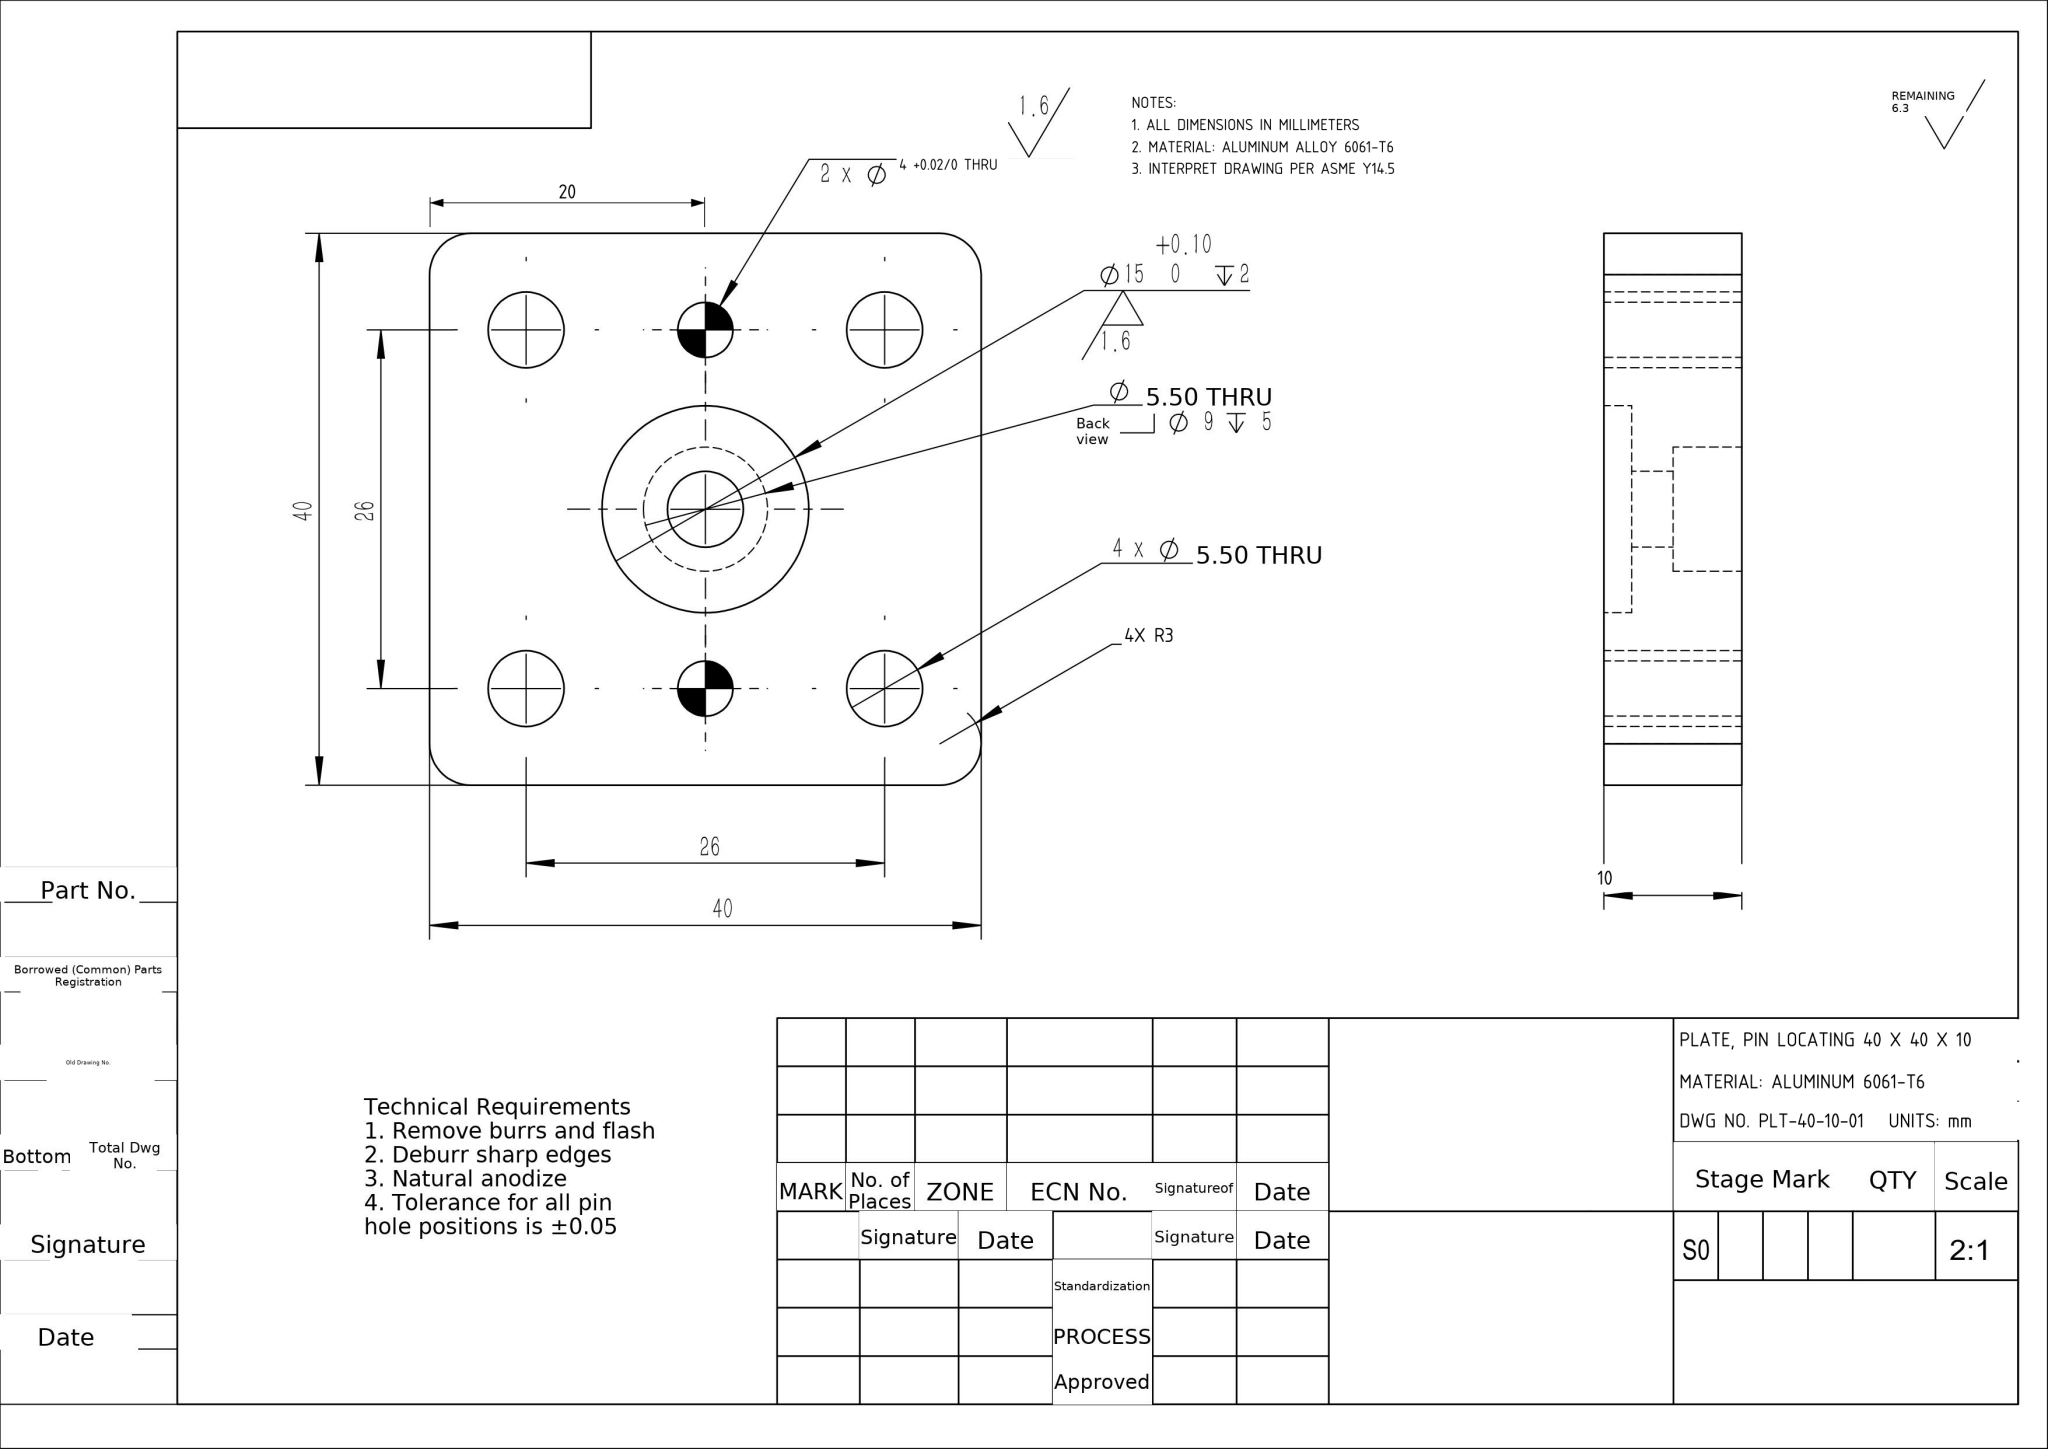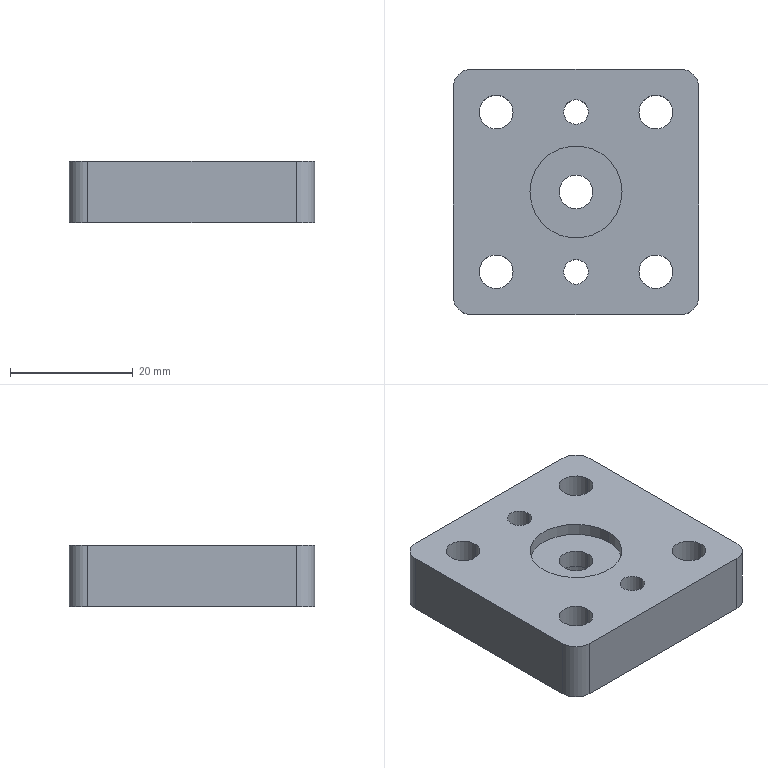Part | NX | mm | 1 solid | 30 faces | box 40 x 40 x 10 mm | volume 13978 mm3 | cylinder 22 | plane 8 | commonest cylinder face diameters 5.5 x10 4 x4 6 x4 15 x2 9 x2